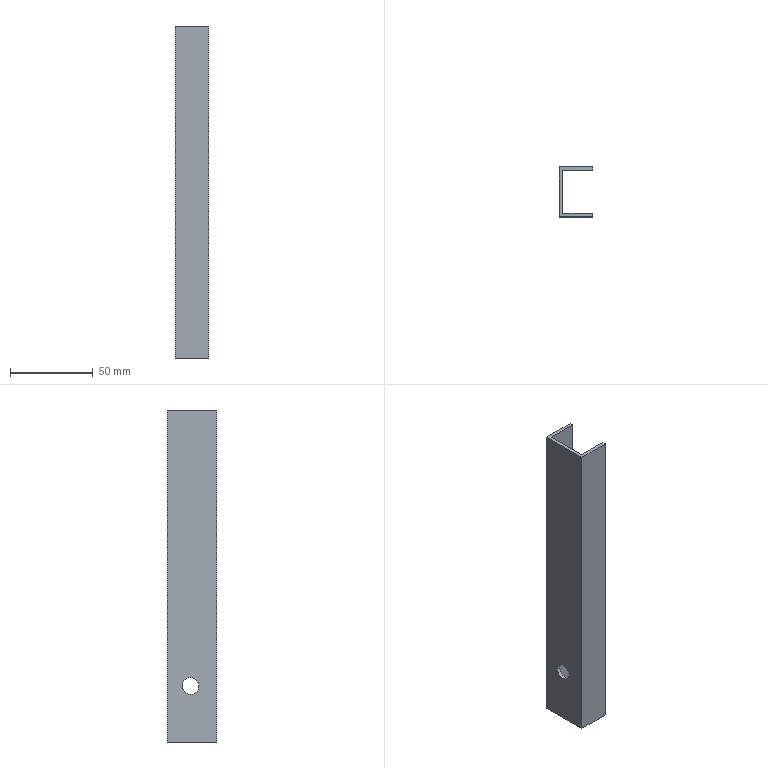Component | SolidWorks | Copy_of_Part3-29 | 1 solid | 12 faces | box 20 x 30 x 200 mm | volume 26243 mm3 | plane 10 | cylinder 2 | commonest cylinder face diameters 10 x2
STEP:
#1=COLOUR_RGB('',0.7922,0.8196,0.9333);
#2=FILL_AREA_STYLE_COLOUR('',#1);
#3=FILL_AREA_STYLE('',(#2));
#4=SURFACE_STYLE_FILL_AREA(#3);
#5=SURFACE_SIDE_STYLE('',(#4));
#6=SURFACE_STYLE_USAGE(.BOTH.,#5);
#7=PRESENTATION_STYLE_ASSIGNMENT((#6));
#8=CARTESIAN_POINT('',(-5.906,8.499,-95.96));
#9=VERTEX_POINT('',#8);
#10=CARTESIAN_POINT('',(-5.906,8.499,-95.566));
#11=VERTEX_POINT('',#10);
#12=CARTESIAN_POINT('',(-5.906,8.499,-95.763));
#13=DIRECTION('',(-1.,-0.,0.));
#14=DIRECTION('',(0.,0.,1.));
#15=AXIS2_PLACEMENT_3D('',#12,#13,#14);
#16=CIRCLE('',#15,0.1969);
#17=EDGE_CURVE('',#9,#11,#16,.T.);
#18=ORIENTED_EDGE('',*,*,#17,.F.);
#19=CARTESIAN_POINT('',(-5.984,8.499,-95.96));
#20=VERTEX_POINT('',#19);
#21=CARTESIAN_POINT('',(-5.197,8.499,-95.96));
#22=DIRECTION('',(-1.,-0.,0.));
#23=VECTOR('',#22,39.37);
#24=LINE('',#21,#23);
#25=EDGE_CURVE('',#9,#20,#24,.T.);
#26=ORIENTED_EDGE('',*,*,#25,.T.);
#27=CARTESIAN_POINT('',(-5.984,8.499,-95.566));
#28=VERTEX_POINT('',#27);
#29=CARTESIAN_POINT('',(-5.984,8.499,-95.96));
#30=CARTESIAN_POINT('',(-5.984,8.473,-95.96));
#31=CARTESIAN_POINT('',(-5.984,8.448,-95.954));
#32=CARTESIAN_POINT('',(-5.984,8.4,-95.935));
#33=CARTESIAN_POINT('',(-5.984,8.378,-95.92));
#34=CARTESIAN_POINT('',(-5.984,8.342,-95.884));
#35=CARTESIAN_POINT('',(-5.984,8.327,-95.862));
#36=CARTESIAN_POINT('',(-5.984,8.307,-95.814));
#37=CARTESIAN_POINT('',(-5.984,8.302,-95.788));
#38=CARTESIAN_POINT('',(-5.984,8.302,-95.737));
#39=CARTESIAN_POINT('',(-5.984,8.307,-95.711));
#40=CARTESIAN_POINT('',(-5.984,8.327,-95.664));
#41=CARTESIAN_POINT('',(-5.984,8.342,-95.642));
#42=CARTESIAN_POINT('',(-5.984,8.378,-95.605));
#43=CARTESIAN_POINT('',(-5.984,8.4,-95.591));
#44=CARTESIAN_POINT('',(-5.984,8.448,-95.571));
#45=CARTESIAN_POINT('',(-5.984,8.473,-95.566));
#46=CARTESIAN_POINT('',(-5.984,8.499,-95.566));
#47=B_SPLINE_CURVE_WITH_KNOTS('',3,(#29,#30,#31,#32,#33,#34,#35,#36,#37,#38,#39,#40,#41,#42,#43,#44,#45,#46),.UNSPECIFIED.,.F.,.F.,(4,2,2,2,2,2,2,2,4),(0.5,0.5625,0.625,0.6875,0.75,0.8125,0.875,0.9375,1.),.UNSPECIFIED.);
#48=EDGE_CURVE('',#20,#28,#47,.T.);
#49=ORIENTED_EDGE('',*,*,#48,.T.);
#50=CARTESIAN_POINT('',(-5.197,8.499,-95.566));
#51=DIRECTION('',(-1.,-0.,0.));
#52=VECTOR('',#51,39.37);
#53=LINE('',#50,#52);
#54=EDGE_CURVE('',#11,#28,#53,.T.);
#55=ORIENTED_EDGE('',*,*,#54,.F.);
#56=EDGE_LOOP('',(#18,#26,#49,#55));
#57=FACE_OUTER_BOUND('',#56,.T.);
#58=CARTESIAN_POINT('',(-5.197,8.499,-95.763));
#59=DIRECTION('',(-1.,-0.,0.));
#60=DIRECTION('',(0.,0.,1.));
#61=AXIS2_PLACEMENT_3D('',#58,#59,#60);
#62=CYLINDRICAL_SURFACE('',#61,0.1969);
#63=ADVANCED_FACE('',(#57),#62,.F.);
#64=CARTESIAN_POINT('',(-5.906,7.953,-89.216));
#65=VERTEX_POINT('',#64);
#66=CARTESIAN_POINT('',(-5.197,7.953,-89.216));
#67=VERTEX_POINT('',#66);
#68=CARTESIAN_POINT('',(-5.984,7.953,-89.216));
#69=DIRECTION('',(1.,-0.,-0.));
#70=VECTOR('',#69,39.37);
#71=LINE('',#68,#70);
#72=EDGE_CURVE('',#65,#67,#71,.T.);
#73=ORIENTED_EDGE('',*,*,#72,.T.);
#74=CARTESIAN_POINT('',(-5.197,7.953,-97.09));
#75=VERTEX_POINT('',#74);
#76=CARTESIAN_POINT('',(-5.197,7.953,-97.09));
#77=DIRECTION('',(0.,0.,1.));
#78=VECTOR('',#77,39.37);
#79=LINE('',#76,#78);
#80=EDGE_CURVE('',#75,#67,#79,.T.);
#81=ORIENTED_EDGE('',*,*,#80,.F.);
#82=CARTESIAN_POINT('',(-5.906,7.953,-97.09));
#83=VERTEX_POINT('',#82);
#84=CARTESIAN_POINT('',(-5.984,7.953,-97.09));
#85=DIRECTION('',(1.,-0.,-0.));
#86=VECTOR('',#85,39.37);
#87=LINE('',#84,#86);
#88=EDGE_CURVE('',#83,#75,#87,.T.);
#89=ORIENTED_EDGE('',*,*,#88,.F.);
#90=CARTESIAN_POINT('',(-5.906,7.953,-97.09));
#91=DIRECTION('',(0.,0.,1.));
#92=VECTOR('',#91,39.37);
#93=LINE('',#90,#92);
#94=EDGE_CURVE('',#83,#65,#93,.T.);
#95=ORIENTED_EDGE('',*,*,#94,.T.);
#96=EDGE_LOOP('',(#73,#81,#89,#95));
#97=FACE_OUTER_BOUND('',#96,.T.);
#98=CARTESIAN_POINT('',(-5.984,7.953,-97.09));
#99=DIRECTION('',(-0.,-1.,-0.));
#100=DIRECTION('',(-1.,0.,0.));
#101=AXIS2_PLACEMENT_3D('',#98,#99,#100);
#102=PLANE('',#101);
#103=ADVANCED_FACE('',(#97),#102,.F.);
#104=CARTESIAN_POINT('',(-5.197,7.874,-89.216));
#105=VERTEX_POINT('',#104);
#106=CARTESIAN_POINT('',(-5.197,7.874,-89.216));
#107=DIRECTION('',(0.,1.,0.));
#108=VECTOR('',#107,39.37);
#109=LINE('',#106,#108);
#110=EDGE_CURVE('',#105,#67,#109,.T.);
#111=ORIENTED_EDGE('',*,*,#110,.F.);
#112=CARTESIAN_POINT('',(-5.197,7.874,-97.09));
#113=VERTEX_POINT('',#112);
#114=CARTESIAN_POINT('',(-5.197,7.874,-97.09));
#115=DIRECTION('',(0.,0.,1.));
#116=VECTOR('',#115,39.37);
#117=LINE('',#114,#116);
#118=EDGE_CURVE('',#113,#105,#117,.T.);
#119=ORIENTED_EDGE('',*,*,#118,.F.);
#120=CARTESIAN_POINT('',(-5.197,7.874,-97.09));
#121=DIRECTION('',(0.,1.,0.));
#122=VECTOR('',#121,39.37);
#123=LINE('',#120,#122);
#124=EDGE_CURVE('',#113,#75,#123,.T.);
#125=ORIENTED_EDGE('',*,*,#124,.T.);
#126=ORIENTED_EDGE('',*,*,#80,.T.);
#127=EDGE_LOOP('',(#111,#119,#125,#126));
#128=FACE_OUTER_BOUND('',#127,.T.);
#129=CARTESIAN_POINT('',(-5.197,7.874,-97.09));
#130=DIRECTION('',(1.,0.,-0.));
#131=DIRECTION('',(-0.,-0.,-1.));
#132=AXIS2_PLACEMENT_3D('',#129,#130,#131);
#133=PLANE('',#132);
#134=ADVANCED_FACE('',(#128),#133,.T.);
#135=CARTESIAN_POINT('',(-5.984,7.874,-89.216));
#136=VERTEX_POINT('',#135);
#137=CARTESIAN_POINT('',(-5.984,7.874,-89.216));
#138=DIRECTION('',(1.,-0.,-0.));
#139=VECTOR('',#138,39.37);
#140=LINE('',#137,#139);
#141=EDGE_CURVE('',#136,#105,#140,.T.);
#142=ORIENTED_EDGE('',*,*,#141,.F.);
#143=CARTESIAN_POINT('',(-5.984,7.874,-97.09));
#144=VERTEX_POINT('',#143);
#145=CARTESIAN_POINT('',(-5.984,7.874,-97.09));
#146=DIRECTION('',(0.,0.,1.));
#147=VECTOR('',#146,39.37);
#148=LINE('',#145,#147);
#149=EDGE_CURVE('',#144,#136,#148,.T.);
#150=ORIENTED_EDGE('',*,*,#149,.F.);
#151=CARTESIAN_POINT('',(-5.984,7.874,-97.09));
#152=DIRECTION('',(1.,-0.,-0.));
#153=VECTOR('',#152,39.37);
#154=LINE('',#151,#153);
#155=EDGE_CURVE('',#144,#113,#154,.T.);
#156=ORIENTED_EDGE('',*,*,#155,.T.);
#157=ORIENTED_EDGE('',*,*,#118,.T.);
#158=EDGE_LOOP('',(#142,#150,#156,#157));
#159=FACE_OUTER_BOUND('',#158,.T.);
#160=CARTESIAN_POINT('',(-5.984,7.874,-97.09));
#161=DIRECTION('',(-0.,-1.,-0.));
#162=DIRECTION('',(-1.,0.,0.));
#163=AXIS2_PLACEMENT_3D('',#160,#161,#162);
#164=PLANE('',#163);
#165=ADVANCED_FACE('',(#159),#164,.T.);
#166=CARTESIAN_POINT('',(-5.984,8.499,-95.566));
#167=CARTESIAN_POINT('',(-5.984,8.525,-95.566));
#168=CARTESIAN_POINT('',(-5.984,8.551,-95.571));
#169=CARTESIAN_POINT('',(-5.984,8.598,-95.591));
#170=CARTESIAN_POINT('',(-5.984,8.62,-95.605));
#171=CARTESIAN_POINT('',(-5.984,8.656,-95.642));
#172=CARTESIAN_POINT('',(-5.984,8.671,-95.664));
#173=CARTESIAN_POINT('',(-5.984,8.691,-95.711));
#174=CARTESIAN_POINT('',(-5.984,8.696,-95.737));
#175=CARTESIAN_POINT('',(-5.984,8.696,-95.788));
#176=CARTESIAN_POINT('',(-5.984,8.691,-95.814));
#177=CARTESIAN_POINT('',(-5.984,8.671,-95.862));
#178=CARTESIAN_POINT('',(-5.984,8.656,-95.884));
#179=CARTESIAN_POINT('',(-5.984,8.62,-95.92));
#180=CARTESIAN_POINT('',(-5.984,8.598,-95.935));
#181=CARTESIAN_POINT('',(-5.984,8.551,-95.954));
#182=CARTESIAN_POINT('',(-5.984,8.525,-95.96));
#183=CARTESIAN_POINT('',(-5.984,8.499,-95.96));
#184=B_SPLINE_CURVE_WITH_KNOTS('',3,(#166,#167,#168,#169,#170,#171,#172,#173,#174,#175,#176,#177,#178,#179,#180,#181,#182,#183),.UNSPECIFIED.,.F.,.F.,(4,2,2,2,2,2,2,2,4),(0.,0.0625,0.125,0.1875,0.25,0.3125,0.375,0.4375,0.5),.UNSPECIFIED.);
#185=EDGE_CURVE('',#28,#20,#184,.T.);
#186=ORIENTED_EDGE('',*,*,#185,.F.);
#187=ORIENTED_EDGE('',*,*,#48,.F.);
#188=EDGE_LOOP('',(#186,#187));
#189=FACE_BOUND('',#188,.T.);
#190=CARTESIAN_POINT('',(-5.984,9.055,-89.216));
#191=VERTEX_POINT('',#190);
#192=CARTESIAN_POINT('',(-5.984,7.874,-89.216));
#193=DIRECTION('',(-0.,-1.,-0.));
#194=VECTOR('',#193,39.37);
#195=LINE('',#192,#194);
#196=EDGE_CURVE('',#191,#136,#195,.T.);
#197=ORIENTED_EDGE('',*,*,#196,.F.);
#198=CARTESIAN_POINT('',(-5.984,9.055,-97.09));
#199=VERTEX_POINT('',#198);
#200=CARTESIAN_POINT('',(-5.984,9.055,-97.09));
#201=DIRECTION('',(0.,0.,1.));
#202=VECTOR('',#201,39.37);
#203=LINE('',#200,#202);
#204=EDGE_CURVE('',#199,#191,#203,.T.);
#205=ORIENTED_EDGE('',*,*,#204,.F.);
#206=CARTESIAN_POINT('',(-5.984,7.874,-97.09));
#207=DIRECTION('',(-0.,-1.,-0.));
#208=VECTOR('',#207,39.37);
#209=LINE('',#206,#208);
#210=EDGE_CURVE('',#199,#144,#209,.T.);
#211=ORIENTED_EDGE('',*,*,#210,.T.);
#212=ORIENTED_EDGE('',*,*,#149,.T.);
#213=EDGE_LOOP('',(#197,#205,#211,#212));
#214=FACE_OUTER_BOUND('',#213,.T.);
#215=CARTESIAN_POINT('',(-5.984,7.874,-97.09));
#216=DIRECTION('',(-1.,-0.,0.));
#217=DIRECTION('',(0.,0.,1.));
#218=AXIS2_PLACEMENT_3D('',#215,#216,#217);
#219=PLANE('',#218);
#220=ADVANCED_FACE('',(#189,#214),#219,.T.);
#221=CARTESIAN_POINT('',(-5.197,9.055,-89.216));
#222=VERTEX_POINT('',#221);
#223=CARTESIAN_POINT('',(-5.984,9.055,-89.216));
#224=DIRECTION('',(-1.,-0.,0.));
#225=VECTOR('',#224,39.37);
#226=LINE('',#223,#225);
#227=EDGE_CURVE('',#222,#191,#226,.T.);
#228=ORIENTED_EDGE('',*,*,#227,.F.);
#229=CARTESIAN_POINT('',(-5.197,9.055,-97.09));
#230=VERTEX_POINT('',#229);
#231=CARTESIAN_POINT('',(-5.197,9.055,-97.09));
#232=DIRECTION('',(0.,0.,1.));
#233=VECTOR('',#232,39.37);
#234=LINE('',#231,#233);
#235=EDGE_CURVE('',#230,#222,#234,.T.);
#236=ORIENTED_EDGE('',*,*,#235,.F.);
#237=CARTESIAN_POINT('',(-5.984,9.055,-97.09));
#238=DIRECTION('',(-1.,-0.,0.));
#239=VECTOR('',#238,39.37);
#240=LINE('',#237,#239);
#241=EDGE_CURVE('',#230,#199,#240,.T.);
#242=ORIENTED_EDGE('',*,*,#241,.T.);
#243=ORIENTED_EDGE('',*,*,#204,.T.);
#244=EDGE_LOOP('',(#228,#236,#242,#243));
#245=FACE_OUTER_BOUND('',#244,.T.);
#246=CARTESIAN_POINT('',(-5.984,9.055,-97.09));
#247=DIRECTION('',(0.,1.,-0.));
#248=DIRECTION('',(-0.,-0.,-1.));
#249=AXIS2_PLACEMENT_3D('',#246,#247,#248);
#250=PLANE('',#249);
#251=ADVANCED_FACE('',(#245),#250,.T.);
#252=CARTESIAN_POINT('',(-5.197,8.976,-89.216));
#253=VERTEX_POINT('',#252);
#254=CARTESIAN_POINT('',(-5.197,8.976,-89.216));
#255=DIRECTION('',(0.,1.,0.));
#256=VECTOR('',#255,39.37);
#257=LINE('',#254,#256);
#258=EDGE_CURVE('',#253,#222,#257,.T.);
#259=ORIENTED_EDGE('',*,*,#258,.F.);
#260=CARTESIAN_POINT('',(-5.197,8.976,-97.09));
#261=VERTEX_POINT('',#260);
#262=CARTESIAN_POINT('',(-5.197,8.976,-97.09));
#263=DIRECTION('',(0.,0.,1.));
#264=VECTOR('',#263,39.37);
#265=LINE('',#262,#264);
#266=EDGE_CURVE('',#261,#253,#265,.T.);
#267=ORIENTED_EDGE('',*,*,#266,.F.);
#268=CARTESIAN_POINT('',(-5.197,8.976,-97.09));
#269=DIRECTION('',(0.,1.,0.));
#270=VECTOR('',#269,39.37);
#271=LINE('',#268,#270);
#272=EDGE_CURVE('',#261,#230,#271,.T.);
#273=ORIENTED_EDGE('',*,*,#272,.T.);
#274=ORIENTED_EDGE('',*,*,#235,.T.);
#275=EDGE_LOOP('',(#259,#267,#273,#274));
#276=FACE_OUTER_BOUND('',#275,.T.);
#277=CARTESIAN_POINT('',(-5.197,8.976,-97.09));
#278=DIRECTION('',(1.,0.,-0.));
#279=DIRECTION('',(-0.,-0.,-1.));
#280=AXIS2_PLACEMENT_3D('',#277,#278,#279);
#281=PLANE('',#280);
#282=ADVANCED_FACE('',(#276),#281,.T.);
#283=CARTESIAN_POINT('',(-5.906,8.976,-89.216));
#284=VERTEX_POINT('',#283);
#285=CARTESIAN_POINT('',(-5.984,8.976,-89.216));
#286=DIRECTION('',(-1.,-0.,0.));
#287=VECTOR('',#286,39.37);
#288=LINE('',#285,#287);
#289=EDGE_CURVE('',#253,#284,#288,.T.);
#290=ORIENTED_EDGE('',*,*,#289,.T.);
#291=CARTESIAN_POINT('',(-5.906,8.976,-97.09));
#292=VERTEX_POINT('',#291);
#293=CARTESIAN_POINT('',(-5.906,8.976,-97.09));
#294=DIRECTION('',(0.,0.,1.));
#295=VECTOR('',#294,39.37);
#296=LINE('',#293,#295);
#297=EDGE_CURVE('',#292,#284,#296,.T.);
#298=ORIENTED_EDGE('',*,*,#297,.F.);
#299=CARTESIAN_POINT('',(-5.984,8.976,-97.09));
#300=DIRECTION('',(-1.,-0.,0.));
#301=VECTOR('',#300,39.37);
#302=LINE('',#299,#301);
#303=EDGE_CURVE('',#261,#292,#302,.T.);
#304=ORIENTED_EDGE('',*,*,#303,.F.);
#305=ORIENTED_EDGE('',*,*,#266,.T.);
#306=EDGE_LOOP('',(#290,#298,#304,#305));
#307=FACE_OUTER_BOUND('',#306,.T.);
#308=CARTESIAN_POINT('',(-5.984,8.976,-97.09));
#309=DIRECTION('',(0.,1.,-0.));
#310=DIRECTION('',(-0.,-0.,-1.));
#311=AXIS2_PLACEMENT_3D('',#308,#309,#310);
#312=PLANE('',#311);
#313=ADVANCED_FACE('',(#307),#312,.F.);
#314=CARTESIAN_POINT('',(-5.906,8.499,-95.763));
#315=DIRECTION('',(-1.,-0.,0.));
#316=DIRECTION('',(0.,0.,1.));
#317=AXIS2_PLACEMENT_3D('',#314,#315,#316);
#318=CIRCLE('',#317,0.1969);
#319=EDGE_CURVE('',#11,#9,#318,.T.);
#320=ORIENTED_EDGE('',*,*,#319,.T.);
#321=ORIENTED_EDGE('',*,*,#17,.T.);
#322=EDGE_LOOP('',(#320,#321));
#323=FACE_BOUND('',#322,.T.);
#324=CARTESIAN_POINT('',(-5.906,7.874,-89.216));
#325=DIRECTION('',(-0.,-1.,-0.));
#326=VECTOR('',#325,39.37);
#327=LINE('',#324,#326);
#328=EDGE_CURVE('',#284,#65,#327,.T.);
#329=ORIENTED_EDGE('',*,*,#328,.T.);
#330=ORIENTED_EDGE('',*,*,#94,.F.);
#331=CARTESIAN_POINT('',(-5.906,7.874,-97.09));
#332=DIRECTION('',(-0.,-1.,-0.));
#333=VECTOR('',#332,39.37);
#334=LINE('',#331,#333);
#335=EDGE_CURVE('',#292,#83,#334,.T.);
#336=ORIENTED_EDGE('',*,*,#335,.F.);
#337=ORIENTED_EDGE('',*,*,#297,.T.);
#338=EDGE_LOOP('',(#329,#330,#336,#337));
#339=FACE_OUTER_BOUND('',#338,.T.);
#340=CARTESIAN_POINT('',(-5.906,7.874,-97.09));
#341=DIRECTION('',(-1.,-0.,0.));
#342=DIRECTION('',(0.,0.,1.));
#343=AXIS2_PLACEMENT_3D('',#340,#341,#342);
#344=PLANE('',#343);
#345=ADVANCED_FACE('',(#323,#339),#344,.F.);
#346=ORIENTED_EDGE('',*,*,#88,.T.);
#347=ORIENTED_EDGE('',*,*,#124,.F.);
#348=ORIENTED_EDGE('',*,*,#155,.F.);
#349=ORIENTED_EDGE('',*,*,#210,.F.);
#350=ORIENTED_EDGE('',*,*,#241,.F.);
#351=ORIENTED_EDGE('',*,*,#272,.F.);
#352=ORIENTED_EDGE('',*,*,#303,.T.);
#353=ORIENTED_EDGE('',*,*,#335,.T.);
#354=EDGE_LOOP('',(#346,#347,#348,#349,#350,#351,#352,#353));
#355=FACE_OUTER_BOUND('',#354,.T.);
#356=CARTESIAN_POINT('',(-5.984,8.43,-97.09));
#357=DIRECTION('',(0.,0.,1.));
#358=DIRECTION('',(1.,0.,-0.));
#359=AXIS2_PLACEMENT_3D('',#356,#357,#358);
#360=PLANE('',#359);
#361=ADVANCED_FACE('',(#355),#360,.F.);
#362=ORIENTED_EDGE('',*,*,#72,.F.);
#363=ORIENTED_EDGE('',*,*,#328,.F.);
#364=ORIENTED_EDGE('',*,*,#289,.F.);
#365=ORIENTED_EDGE('',*,*,#258,.T.);
#366=ORIENTED_EDGE('',*,*,#227,.T.);
#367=ORIENTED_EDGE('',*,*,#196,.T.);
#368=ORIENTED_EDGE('',*,*,#141,.T.);
#369=ORIENTED_EDGE('',*,*,#110,.T.);
#370=EDGE_LOOP('',(#362,#363,#364,#365,#366,#367,#368,#369));
#371=FACE_OUTER_BOUND('',#370,.T.);
#372=CARTESIAN_POINT('',(-5.984,8.43,-89.216));
#373=DIRECTION('',(0.,0.,1.));
#374=DIRECTION('',(1.,0.,-0.));
#375=AXIS2_PLACEMENT_3D('',#372,#373,#374);
#376=PLANE('',#375);
#377=ADVANCED_FACE('',(#371),#376,.T.);
#378=ORIENTED_EDGE('',*,*,#25,.F.);
#379=ORIENTED_EDGE('',*,*,#319,.F.);
#380=ORIENTED_EDGE('',*,*,#54,.T.);
#381=ORIENTED_EDGE('',*,*,#185,.T.);
#382=EDGE_LOOP('',(#378,#379,#380,#381));
#383=FACE_OUTER_BOUND('',#382,.T.);
#384=CARTESIAN_POINT('',(-5.197,8.499,-95.763));
#385=DIRECTION('',(-1.,-0.,0.));
#386=DIRECTION('',(0.,0.,1.));
#387=AXIS2_PLACEMENT_3D('',#384,#385,#386);
#388=CYLINDRICAL_SURFACE('',#387,0.1969);
#389=ADVANCED_FACE('',(#383),#388,.F.);
#390=CLOSED_SHELL('',(#63,#103,#134,#165,#220,#251,#282,#313,#345,#361,#377,#389));
#391=MANIFOLD_SOLID_BREP('',#390);
#392=STYLED_ITEM('',(#7),#391);
#393=(LENGTH_UNIT()NAMED_UNIT(*)SI_UNIT($,.METRE.));
#394=LENGTH_MEASURE_WITH_UNIT(LENGTH_MEASURE(0.0254),#393);
#395=DIMENSIONAL_EXPONENTS(1.,0.,0.,0.,0.,0.,0.);
#396=(CONVERSION_BASED_UNIT('',#394)LENGTH_UNIT()NAMED_UNIT(#395));
#397=UNCERTAINTY_MEASURE_WITH_UNIT(LENGTH_MEASURE(0.00001),#396,'','');
#398=(NAMED_UNIT(*)PLANE_ANGLE_UNIT()SI_UNIT($,.RADIAN.));
#399=(NAMED_UNIT(*)SI_UNIT($,.STERADIAN.)SOLID_ANGLE_UNIT());
#400=(GEOMETRIC_REPRESENTATION_CONTEXT(3)GLOBAL_UNCERTAINTY_ASSIGNED_CONTEXT((#397))GLOBAL_UNIT_ASSIGNED_CONTEXT((#396,#398,#399))REPRESENTATION_CONTEXT('',''));
#401=MECHANICAL_DESIGN_GEOMETRIC_PRESENTATION_REPRESENTATION('',(#392),#400);
#402=PRESENTATION_LAYER_ASSIGNMENT('','',(#392));
#403=CARTESIAN_POINT('',(0.,0.,0.));
#404=DIRECTION('',(0.,0.,1.));
#405=DIRECTION('',(1.,0.,0.));
#406=AXIS2_PLACEMENT_3D('',#403,#404,#405);
#407=(LENGTH_UNIT()NAMED_UNIT(*)SI_UNIT($,.METRE.));
#408=LENGTH_MEASURE_WITH_UNIT(LENGTH_MEASURE(0.0254),#407);
#409=DIMENSIONAL_EXPONENTS(1.,0.,0.,0.,0.,0.,0.);
#410=(CONVERSION_BASED_UNIT('',#408)LENGTH_UNIT()NAMED_UNIT(#409));
#411=UNCERTAINTY_MEASURE_WITH_UNIT(LENGTH_MEASURE(0.00001),#410,'','');
#412=(NAMED_UNIT(*)PLANE_ANGLE_UNIT()SI_UNIT($,.RADIAN.));
#413=(NAMED_UNIT(*)SI_UNIT($,.STERADIAN.)SOLID_ANGLE_UNIT());
#414=(GEOMETRIC_REPRESENTATION_CONTEXT(3)GLOBAL_UNCERTAINTY_ASSIGNED_CONTEXT((#411))GLOBAL_UNIT_ASSIGNED_CONTEXT((#410,#412,#413))REPRESENTATION_CONTEXT('',''));
#415=ADVANCED_BREP_SHAPE_REPRESENTATION('',(#391,#406),#414);